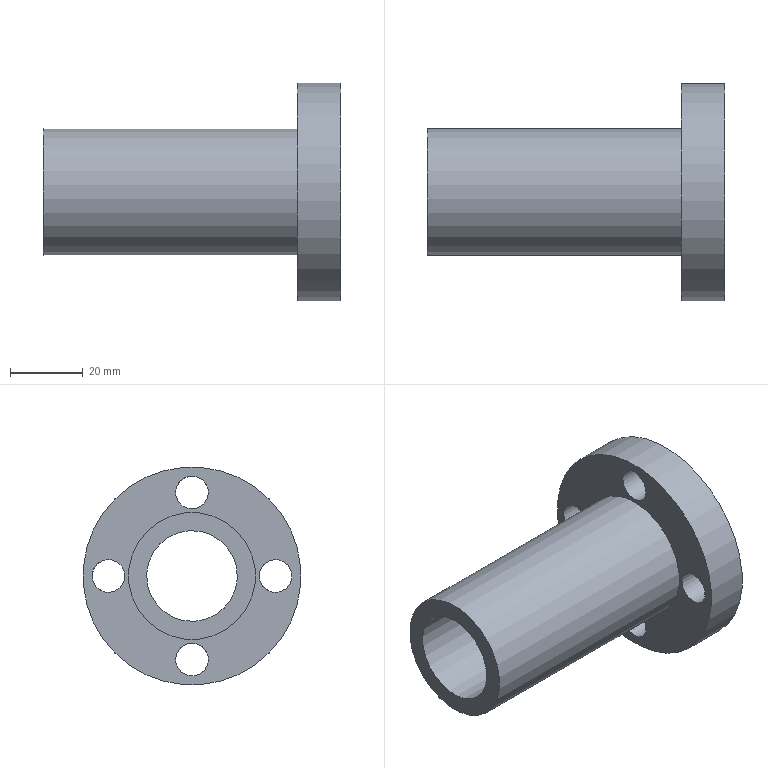Component | NX | LEADSCREW_NUT | 1 solid | 10 faces | box 82 x 60 x 60 mm | volume 57972 mm3 | cylinder 7 | plane 3 | commonest cylinder face diameters 9 x4 25 x1 60 x1 35 x1
STEP:
#1=CARTESIAN_POINT('',(0.,0.,0.));
#2=DIRECTION('',(0.,0.,1.));
#3=DIRECTION('',(1.,0.,0.));
#4=AXIS2_PLACEMENT_3D('',#1,#2,#3);
#5=CARTESIAN_POINT('',(639.189,-141.463,-1564.161));
#6=VERTEX_POINT('',#5);
#7=CARTESIAN_POINT('',(639.189,-150.302,-1573.));
#8=DIRECTION('',(-1.,0.,0.));
#9=DIRECTION('',(0.,0.7071,0.7071));
#10=AXIS2_PLACEMENT_3D('',#7,#8,#9);
#11=CIRCLE('',#10,12.5);
#12=CARTESIAN_POINT('',(639.189,-137.927,-1560.626));
#13=DIRECTION('',(1.,0.,0.));
#14=DIRECTION('',(0.,-0.7071,-0.7071));
#15=AXIS2_PLACEMENT_3D('',#12,#13,#14);
#16=PLANE('',#15);
#17=CARTESIAN_POINT('',(5.,-0.));
#18=CARTESIAN_POINT('',(5.,21.651));
#19=CARTESIAN_POINT('',(23.75,10.825));
#20=CARTESIAN_POINT('',(42.5,-0.));
#21=CARTESIAN_POINT('',(23.75,-10.825));
#22=CARTESIAN_POINT('',(5.,-21.651));
#23=CARTESIAN_POINT('',(5.,-0.));
#24=(BOUNDED_CURVE()B_SPLINE_CURVE(2,(#17,#18,#19,#20,#21,#22,#23),.UNSPECIFIED.,.T.,.F.)B_SPLINE_CURVE_WITH_KNOTS((1,2,2,2,2,1),(-2.094,0.,2.094,4.189,6.283,8.378),.UNSPECIFIED.)CURVE()GEOMETRIC_REPRESENTATION_ITEM()RATIONAL_B_SPLINE_CURVE((1.,0.5,1.,0.5,1.,0.5,1.))REPRESENTATION_ITEM(''));
#25=(GEOMETRIC_REPRESENTATION_CONTEXT(2)PARAMETRIC_REPRESENTATION_CONTEXT()REPRESENTATION_CONTEXT('',''));
#26=DEFINITIONAL_REPRESENTATION('',(#24),#25);
#27=PCURVE('',#16,#26);
#28=CARTESIAN_POINT('',(639.189,-150.302,-1573.));
#29=DIRECTION('',(-1.,0.,0.));
#30=DIRECTION('',(0.,0.7071,0.7071));
#31=AXIS2_PLACEMENT_3D('',#28,#29,#30);
#32=CYLINDRICAL_SURFACE('',#31,12.5);
#33=CARTESIAN_POINT('',(0.,0.));
#34=DIRECTION('',(1.,0.));
#35=VECTOR('',#34,1.);
#36=LINE('',#33,#35);
#37=(GEOMETRIC_REPRESENTATION_CONTEXT(2)PARAMETRIC_REPRESENTATION_CONTEXT()REPRESENTATION_CONTEXT('',''));
#38=DEFINITIONAL_REPRESENTATION('',(#36),#37);
#39=PCURVE('',#32,#38);
#40=SURFACE_CURVE('',#11,(#27,#39),.PCURVE_S1.);
#41=EDGE_CURVE('',#6,#6,#40,.T.);
#42=ORIENTED_EDGE('',*,*,#41,.F.);
#43=EDGE_LOOP('',(#42));
#44=FACE_BOUND('',#43,.T.);
#45=CARTESIAN_POINT('',(639.189,-137.927,-1560.626));
#46=VERTEX_POINT('',#45);
#47=CARTESIAN_POINT('',(639.189,-150.302,-1573.));
#48=DIRECTION('',(-1.,0.,0.));
#49=DIRECTION('',(0.,0.7071,0.7071));
#50=AXIS2_PLACEMENT_3D('',#47,#48,#49);
#51=CIRCLE('',#50,17.5);
#52=CARTESIAN_POINT('',(-0.,-0.));
#53=CARTESIAN_POINT('',(-0.,30.311));
#54=CARTESIAN_POINT('',(26.25,15.155));
#55=CARTESIAN_POINT('',(52.5,-0.));
#56=CARTESIAN_POINT('',(26.25,-15.155));
#57=CARTESIAN_POINT('',(-0.,-30.311));
#58=CARTESIAN_POINT('',(-0.,-0.));
#59=(BOUNDED_CURVE()B_SPLINE_CURVE(2,(#52,#53,#54,#55,#56,#57,#58),.UNSPECIFIED.,.T.,.F.)B_SPLINE_CURVE_WITH_KNOTS((1,2,2,2,2,1),(-2.094,0.,2.094,4.189,6.283,8.378),.UNSPECIFIED.)CURVE()GEOMETRIC_REPRESENTATION_ITEM()RATIONAL_B_SPLINE_CURVE((1.,0.5,1.,0.5,1.,0.5,1.))REPRESENTATION_ITEM(''));
#60=(GEOMETRIC_REPRESENTATION_CONTEXT(2)PARAMETRIC_REPRESENTATION_CONTEXT()REPRESENTATION_CONTEXT('',''));
#61=DEFINITIONAL_REPRESENTATION('',(#59),#60);
#62=PCURVE('',#16,#61);
#63=CARTESIAN_POINT('',(639.189,-150.302,-1573.));
#64=DIRECTION('',(-1.,0.,0.));
#65=DIRECTION('',(0.,0.7071,0.7071));
#66=AXIS2_PLACEMENT_3D('',#63,#64,#65);
#67=CYLINDRICAL_SURFACE('',#66,17.5);
#68=CARTESIAN_POINT('',(0.,0.));
#69=DIRECTION('',(1.,0.));
#70=VECTOR('',#69,1.);
#71=LINE('',#68,#70);
#72=(GEOMETRIC_REPRESENTATION_CONTEXT(2)PARAMETRIC_REPRESENTATION_CONTEXT()REPRESENTATION_CONTEXT('',''));
#73=DEFINITIONAL_REPRESENTATION('',(#71),#72);
#74=PCURVE('',#67,#73);
#75=SURFACE_CURVE('',#51,(#62,#74),.PCURVE_S1.);
#76=EDGE_CURVE('',#46,#46,#75,.T.);
#77=ORIENTED_EDGE('',*,*,#76,.T.);
#78=EDGE_LOOP('',(#77));
#79=FACE_BOUND('',#78,.T.);
#80=ADVANCED_FACE('',(#44,#79),#16,.F.);
#81=CARTESIAN_POINT('',(721.189,-141.463,-1564.161));
#82=VERTEX_POINT('',#81);
#83=CARTESIAN_POINT('',(721.189,-150.302,-1573.));
#84=DIRECTION('',(-1.,0.,0.));
#85=DIRECTION('',(0.,0.7071,0.7071));
#86=AXIS2_PLACEMENT_3D('',#83,#84,#85);
#87=CIRCLE('',#86,12.5);
#88=CARTESIAN_POINT('',(0.,-82.));
#89=DIRECTION('',(1.,0.));
#90=VECTOR('',#89,1.);
#91=LINE('',#88,#90);
#92=(GEOMETRIC_REPRESENTATION_CONTEXT(2)PARAMETRIC_REPRESENTATION_CONTEXT()REPRESENTATION_CONTEXT('',''));
#93=DEFINITIONAL_REPRESENTATION('',(#91),#92);
#94=PCURVE('',#32,#93);
#95=CARTESIAN_POINT('',(721.189,-141.463,-1564.161));
#96=DIRECTION('',(-1.,0.,0.));
#97=DIRECTION('',(0.,0.7071,0.7071));
#98=AXIS2_PLACEMENT_3D('',#95,#96,#97);
#99=PLANE('',#98);
#100=CARTESIAN_POINT('',(-12.5,-0.));
#101=DIRECTION('',(1.,0.));
#102=AXIS2_PLACEMENT_2D('',#100,#101);
#103=CIRCLE('',#102,12.5);
#104=(GEOMETRIC_REPRESENTATION_CONTEXT(2)PARAMETRIC_REPRESENTATION_CONTEXT()REPRESENTATION_CONTEXT('',''));
#105=DEFINITIONAL_REPRESENTATION('',(#103),#104);
#106=PCURVE('',#99,#105);
#107=SURFACE_CURVE('',#87,(#94,#106),.PCURVE_S1.);
#108=EDGE_CURVE('',#82,#82,#107,.T.);
#109=ORIENTED_EDGE('',*,*,#108,.T.);
#110=CARTESIAN_POINT('',(721.189,-141.463,-1564.161));
#111=CARTESIAN_POINT('',(639.189,-141.463,-1564.161));
#112=B_SPLINE_CURVE_WITH_KNOTS('',1,(#110,#111),.UNSPECIFIED.,.F.,.F.,(2,2),(-82.,0.),.PIECEWISE_BEZIER_KNOTS.);
#113=CARTESIAN_POINT('',(6.283,0.));
#114=DIRECTION('',(0.,1.));
#115=VECTOR('',#114,1.);
#116=LINE('',#113,#115);
#117=(GEOMETRIC_REPRESENTATION_CONTEXT(2)PARAMETRIC_REPRESENTATION_CONTEXT()REPRESENTATION_CONTEXT('',''));
#118=DEFINITIONAL_REPRESENTATION('',(#116),#117);
#119=PCURVE('',#32,#118);
#120=CARTESIAN_POINT('',(0.,0.));
#121=DIRECTION('',(0.,1.));
#122=VECTOR('',#121,1.);
#123=LINE('',#120,#122);
#124=(GEOMETRIC_REPRESENTATION_CONTEXT(2)PARAMETRIC_REPRESENTATION_CONTEXT()REPRESENTATION_CONTEXT('',''));
#125=DEFINITIONAL_REPRESENTATION('',(#123),#124);
#126=PCURVE('',#32,#125);
#127=SEAM_CURVE('',#112,(#119,#126),.PCURVE_S1.);
#128=EDGE_CURVE('',#82,#6,#127,.T.);
#129=ORIENTED_EDGE('',*,*,#128,.T.);
#130=ORIENTED_EDGE('',*,*,#41,.F.);
#131=ORIENTED_EDGE('',*,*,#128,.F.);
#132=EDGE_LOOP('',(#109,#129,#130,#131));
#133=FACE_BOUND('',#132,.F.);
#134=ADVANCED_FACE('',(#133),#32,.F.);
#135=CARTESIAN_POINT('',(721.189,-168.802,-1573.));
#136=VERTEX_POINT('',#135);
#137=CARTESIAN_POINT('',(721.189,-176.484,-1576.182));
#138=VERTEX_POINT('',#137);
#139=CARTESIAN_POINT('',(721.189,-173.302,-1573.));
#140=DIRECTION('',(1.,0.,0.));
#141=DIRECTION('',(0.,1.,0.));
#142=AXIS2_PLACEMENT_3D('',#139,#140,#141);
#143=CIRCLE('',#142,4.5);
#144=CARTESIAN_POINT('',(-25.581,-13.081));
#145=CARTESIAN_POINT('',(-20.07,-18.593));
#146=CARTESIAN_POINT('',(-27.599,-20.61));
#147=CARTESIAN_POINT('',(-35.127,-22.627));
#148=CARTESIAN_POINT('',(-33.11,-15.099));
#149=CARTESIAN_POINT('',(-31.093,-7.57));
#150=CARTESIAN_POINT('',(-25.581,-13.081));
#151=(BOUNDED_CURVE()B_SPLINE_CURVE(2,(#144,#145,#146,#147,#148,#149,#150),.UNSPECIFIED.,.T.,.F.)B_SPLINE_CURVE_WITH_KNOTS((1,2,2,2,2,1),(-2.094,0.,2.094,4.189,6.283,8.378),.UNSPECIFIED.)CURVE()GEOMETRIC_REPRESENTATION_ITEM()RATIONAL_B_SPLINE_CURVE((1.,0.5,1.,0.5,1.,0.5,1.))REPRESENTATION_ITEM(''));
#152=(GEOMETRIC_REPRESENTATION_CONTEXT(2)PARAMETRIC_REPRESENTATION_CONTEXT()REPRESENTATION_CONTEXT('',''));
#153=DEFINITIONAL_REPRESENTATION('',(#151),#152);
#154=PCURVE('',#99,#153);
#155=CARTESIAN_POINT('',(704.189,-173.302,-1573.));
#156=DIRECTION('',(1.,0.,0.));
#157=DIRECTION('',(0.,-0.7071,-0.7071));
#158=AXIS2_PLACEMENT_3D('',#155,#156,#157);
#159=CYLINDRICAL_SURFACE('',#158,4.5);
#160=CARTESIAN_POINT('',(2.356,17.));
#161=DIRECTION('',(1.,0.));
#162=VECTOR('',#161,1.);
#163=LINE('',#160,#162);
#164=(GEOMETRIC_REPRESENTATION_CONTEXT(2)PARAMETRIC_REPRESENTATION_CONTEXT()REPRESENTATION_CONTEXT('',''));
#165=DEFINITIONAL_REPRESENTATION('',(#163),#164);
#166=PCURVE('',#159,#165);
#167=SURFACE_CURVE('',#143,(#154,#166),.PCURVE_S1.);
#168=EDGE_CURVE('',#136,#138,#167,.T.);
#169=ORIENTED_EDGE('',*,*,#168,.F.);
#170=CARTESIAN_POINT('',(721.189,-173.302,-1573.));
#171=DIRECTION('',(1.,0.,0.));
#172=DIRECTION('',(0.,1.,0.));
#173=AXIS2_PLACEMENT_3D('',#170,#171,#172);
#174=CIRCLE('',#173,4.5);
#175=CARTESIAN_POINT('',(-25.581,-13.081));
#176=CARTESIAN_POINT('',(-20.07,-18.593));
#177=CARTESIAN_POINT('',(-27.599,-20.61));
#178=CARTESIAN_POINT('',(-35.127,-22.627));
#179=CARTESIAN_POINT('',(-33.11,-15.099));
#180=CARTESIAN_POINT('',(-31.093,-7.57));
#181=CARTESIAN_POINT('',(-25.581,-13.081));
#182=(BOUNDED_CURVE()B_SPLINE_CURVE(2,(#175,#176,#177,#178,#179,#180,#181),.UNSPECIFIED.,.T.,.F.)B_SPLINE_CURVE_WITH_KNOTS((1,2,2,2,2,1),(-2.094,0.,2.094,4.189,6.283,8.378),.UNSPECIFIED.)CURVE()GEOMETRIC_REPRESENTATION_ITEM()RATIONAL_B_SPLINE_CURVE((1.,0.5,1.,0.5,1.,0.5,1.))REPRESENTATION_ITEM(''));
#183=(GEOMETRIC_REPRESENTATION_CONTEXT(2)PARAMETRIC_REPRESENTATION_CONTEXT()REPRESENTATION_CONTEXT('',''));
#184=DEFINITIONAL_REPRESENTATION('',(#182),#183);
#185=PCURVE('',#99,#184);
#186=CARTESIAN_POINT('',(-3.927,17.));
#187=DIRECTION('',(1.,0.));
#188=VECTOR('',#187,1.);
#189=LINE('',#186,#188);
#190=(GEOMETRIC_REPRESENTATION_CONTEXT(2)PARAMETRIC_REPRESENTATION_CONTEXT()REPRESENTATION_CONTEXT('',''));
#191=DEFINITIONAL_REPRESENTATION('',(#189),#190);
#192=PCURVE('',#159,#191);
#193=SURFACE_CURVE('',#174,(#185,#192),.PCURVE_S1.);
#194=EDGE_CURVE('',#138,#136,#193,.T.);
#195=ORIENTED_EDGE('',*,*,#194,.F.);
#196=EDGE_LOOP('',(#169,#195));
#197=FACE_BOUND('',#196,.T.);
#198=CARTESIAN_POINT('',(721.189,-150.302,-1554.5));
#199=VERTEX_POINT('',#198);
#200=CARTESIAN_POINT('',(721.189,-153.484,-1553.182));
#201=VERTEX_POINT('',#200);
#202=CARTESIAN_POINT('',(721.189,-150.302,-1550.));
#203=DIRECTION('',(1.,0.,0.));
#204=DIRECTION('',(0.,0.,-1.));
#205=AXIS2_PLACEMENT_3D('',#202,#203,#204);
#206=CIRCLE('',#205,4.5);
#207=CARTESIAN_POINT('',(0.5815,-13.081));
#208=CARTESIAN_POINT('',(6.093,-7.57));
#209=CARTESIAN_POINT('',(8.11,-15.099));
#210=CARTESIAN_POINT('',(10.127,-22.627));
#211=CARTESIAN_POINT('',(2.599,-20.61));
#212=CARTESIAN_POINT('',(-4.93,-18.593));
#213=CARTESIAN_POINT('',(0.5815,-13.081));
#214=(BOUNDED_CURVE()B_SPLINE_CURVE(2,(#207,#208,#209,#210,#211,#212,#213),.UNSPECIFIED.,.T.,.F.)B_SPLINE_CURVE_WITH_KNOTS((1,2,2,2,2,1),(-2.094,0.,2.094,4.189,6.283,8.378),.UNSPECIFIED.)CURVE()GEOMETRIC_REPRESENTATION_ITEM()RATIONAL_B_SPLINE_CURVE((1.,0.5,1.,0.5,1.,0.5,1.))REPRESENTATION_ITEM(''));
#215=(GEOMETRIC_REPRESENTATION_CONTEXT(2)PARAMETRIC_REPRESENTATION_CONTEXT()REPRESENTATION_CONTEXT('',''));
#216=DEFINITIONAL_REPRESENTATION('',(#214),#215);
#217=PCURVE('',#99,#216);
#218=CARTESIAN_POINT('',(704.189,-150.302,-1550.));
#219=DIRECTION('',(1.,0.,0.));
#220=DIRECTION('',(0.,-0.7071,-0.7071));
#221=AXIS2_PLACEMENT_3D('',#218,#219,#220);
#222=CYLINDRICAL_SURFACE('',#221,4.5);
#223=CARTESIAN_POINT('',(0.7854,17.));
#224=DIRECTION('',(1.,0.));
#225=VECTOR('',#224,1.);
#226=LINE('',#223,#225);
#227=(GEOMETRIC_REPRESENTATION_CONTEXT(2)PARAMETRIC_REPRESENTATION_CONTEXT()REPRESENTATION_CONTEXT('',''));
#228=DEFINITIONAL_REPRESENTATION('',(#226),#227);
#229=PCURVE('',#222,#228);
#230=SURFACE_CURVE('',#206,(#217,#229),.PCURVE_S1.);
#231=EDGE_CURVE('',#199,#201,#230,.T.);
#232=ORIENTED_EDGE('',*,*,#231,.F.);
#233=CARTESIAN_POINT('',(721.189,-150.302,-1550.));
#234=DIRECTION('',(1.,0.,0.));
#235=DIRECTION('',(0.,0.,-1.));
#236=AXIS2_PLACEMENT_3D('',#233,#234,#235);
#237=CIRCLE('',#236,4.5);
#238=CARTESIAN_POINT('',(0.5815,-13.081));
#239=CARTESIAN_POINT('',(6.093,-7.57));
#240=CARTESIAN_POINT('',(8.11,-15.099));
#241=CARTESIAN_POINT('',(10.127,-22.627));
#242=CARTESIAN_POINT('',(2.599,-20.61));
#243=CARTESIAN_POINT('',(-4.93,-18.593));
#244=CARTESIAN_POINT('',(0.5815,-13.081));
#245=(BOUNDED_CURVE()B_SPLINE_CURVE(2,(#238,#239,#240,#241,#242,#243,#244),.UNSPECIFIED.,.T.,.F.)B_SPLINE_CURVE_WITH_KNOTS((1,2,2,2,2,1),(-2.094,0.,2.094,4.189,6.283,8.378),.UNSPECIFIED.)CURVE()GEOMETRIC_REPRESENTATION_ITEM()RATIONAL_B_SPLINE_CURVE((1.,0.5,1.,0.5,1.,0.5,1.))REPRESENTATION_ITEM(''));
#246=(GEOMETRIC_REPRESENTATION_CONTEXT(2)PARAMETRIC_REPRESENTATION_CONTEXT()REPRESENTATION_CONTEXT('',''));
#247=DEFINITIONAL_REPRESENTATION('',(#245),#246);
#248=PCURVE('',#99,#247);
#249=CARTESIAN_POINT('',(-5.498,17.));
#250=DIRECTION('',(1.,0.));
#251=VECTOR('',#250,1.);
#252=LINE('',#249,#251);
#253=(GEOMETRIC_REPRESENTATION_CONTEXT(2)PARAMETRIC_REPRESENTATION_CONTEXT()REPRESENTATION_CONTEXT('',''));
#254=DEFINITIONAL_REPRESENTATION('',(#252),#253);
#255=PCURVE('',#222,#254);
#256=SURFACE_CURVE('',#237,(#248,#255),.PCURVE_S1.);
#257=EDGE_CURVE('',#201,#199,#256,.T.);
#258=ORIENTED_EDGE('',*,*,#257,.F.);
#259=EDGE_LOOP('',(#232,#258));
#260=FACE_BOUND('',#259,.T.);
#261=CARTESIAN_POINT('',(721.189,-150.302,-1591.5));
#262=VERTEX_POINT('',#261);
#263=CARTESIAN_POINT('',(721.189,-153.484,-1599.182));
#264=VERTEX_POINT('',#263);
#265=CARTESIAN_POINT('',(721.189,-150.302,-1596.));
#266=DIRECTION('',(1.,0.,0.));
#267=DIRECTION('',(0.,-0.,1.));
#268=AXIS2_PLACEMENT_3D('',#265,#266,#267);
#269=CIRCLE('',#268,4.5);
#270=CARTESIAN_POINT('',(-25.581,13.081));
#271=CARTESIAN_POINT('',(-31.093,7.57));
#272=CARTESIAN_POINT('',(-33.11,15.099));
#273=CARTESIAN_POINT('',(-35.127,22.627));
#274=CARTESIAN_POINT('',(-27.599,20.61));
#275=CARTESIAN_POINT('',(-20.07,18.593));
#276=CARTESIAN_POINT('',(-25.581,13.081));
#277=(BOUNDED_CURVE()B_SPLINE_CURVE(2,(#270,#271,#272,#273,#274,#275,#276),.UNSPECIFIED.,.T.,.F.)B_SPLINE_CURVE_WITH_KNOTS((1,2,2,2,2,1),(-2.094,0.,2.094,4.189,6.283,8.378),.UNSPECIFIED.)CURVE()GEOMETRIC_REPRESENTATION_ITEM()RATIONAL_B_SPLINE_CURVE((1.,0.5,1.,0.5,1.,0.5,1.))REPRESENTATION_ITEM(''));
#278=(GEOMETRIC_REPRESENTATION_CONTEXT(2)PARAMETRIC_REPRESENTATION_CONTEXT()REPRESENTATION_CONTEXT('',''));
#279=DEFINITIONAL_REPRESENTATION('',(#277),#278);
#280=PCURVE('',#99,#279);
#281=CARTESIAN_POINT('',(704.189,-150.302,-1596.));
#282=DIRECTION('',(1.,0.,0.));
#283=DIRECTION('',(0.,-0.7071,-0.7071));
#284=AXIS2_PLACEMENT_3D('',#281,#282,#283);
#285=CYLINDRICAL_SURFACE('',#284,4.5);
#286=CARTESIAN_POINT('',(3.927,17.));
#287=DIRECTION('',(1.,0.));
#288=VECTOR('',#287,1.);
#289=LINE('',#286,#288);
#290=(GEOMETRIC_REPRESENTATION_CONTEXT(2)PARAMETRIC_REPRESENTATION_CONTEXT()REPRESENTATION_CONTEXT('',''));
#291=DEFINITIONAL_REPRESENTATION('',(#289),#290);
#292=PCURVE('',#285,#291);
#293=SURFACE_CURVE('',#269,(#280,#292),.PCURVE_S1.);
#294=EDGE_CURVE('',#262,#264,#293,.T.);
#295=ORIENTED_EDGE('',*,*,#294,.F.);
#296=CARTESIAN_POINT('',(721.189,-150.302,-1596.));
#297=DIRECTION('',(1.,0.,0.));
#298=DIRECTION('',(0.,-0.,1.));
#299=AXIS2_PLACEMENT_3D('',#296,#297,#298);
#300=CIRCLE('',#299,4.5);
#301=CARTESIAN_POINT('',(-25.581,13.081));
#302=CARTESIAN_POINT('',(-31.093,7.57));
#303=CARTESIAN_POINT('',(-33.11,15.099));
#304=CARTESIAN_POINT('',(-35.127,22.627));
#305=CARTESIAN_POINT('',(-27.599,20.61));
#306=CARTESIAN_POINT('',(-20.07,18.593));
#307=CARTESIAN_POINT('',(-25.581,13.081));
#308=(BOUNDED_CURVE()B_SPLINE_CURVE(2,(#301,#302,#303,#304,#305,#306,#307),.UNSPECIFIED.,.T.,.F.)B_SPLINE_CURVE_WITH_KNOTS((1,2,2,2,2,1),(-2.094,0.,2.094,4.189,6.283,8.378),.UNSPECIFIED.)CURVE()GEOMETRIC_REPRESENTATION_ITEM()RATIONAL_B_SPLINE_CURVE((1.,0.5,1.,0.5,1.,0.5,1.))REPRESENTATION_ITEM(''));
#309=(GEOMETRIC_REPRESENTATION_CONTEXT(2)PARAMETRIC_REPRESENTATION_CONTEXT()REPRESENTATION_CONTEXT('',''));
#310=DEFINITIONAL_REPRESENTATION('',(#308),#309);
#311=PCURVE('',#99,#310);
#312=CARTESIAN_POINT('',(-2.356,17.));
#313=DIRECTION('',(1.,0.));
#314=VECTOR('',#313,1.);
#315=LINE('',#312,#314);
#316=(GEOMETRIC_REPRESENTATION_CONTEXT(2)PARAMETRIC_REPRESENTATION_CONTEXT()REPRESENTATION_CONTEXT('',''));
#317=DEFINITIONAL_REPRESENTATION('',(#315),#316);
#318=PCURVE('',#285,#317);
#319=SURFACE_CURVE('',#300,(#311,#318),.PCURVE_S1.);
#320=EDGE_CURVE('',#264,#262,#319,.T.);
#321=ORIENTED_EDGE('',*,*,#320,.F.);
#322=EDGE_LOOP('',(#295,#321));
#323=FACE_BOUND('',#322,.T.);
#324=CARTESIAN_POINT('',(721.189,-131.802,-1573.));
#325=VERTEX_POINT('',#324);
#326=CARTESIAN_POINT('',(721.189,-130.484,-1576.182));
#327=VERTEX_POINT('',#326);
#328=CARTESIAN_POINT('',(721.189,-127.302,-1573.));
#329=DIRECTION('',(1.,0.,0.));
#330=DIRECTION('',(0.,-1.,0.));
#331=AXIS2_PLACEMENT_3D('',#328,#329,#330);
#332=CIRCLE('',#331,4.5);
#333=CARTESIAN_POINT('',(0.5815,13.081));
#334=CARTESIAN_POINT('',(-4.93,18.593));
#335=CARTESIAN_POINT('',(2.599,20.61));
#336=CARTESIAN_POINT('',(10.127,22.627));
#337=CARTESIAN_POINT('',(8.11,15.099));
#338=CARTESIAN_POINT('',(6.093,7.57));
#339=CARTESIAN_POINT('',(0.5815,13.081));
#340=(BOUNDED_CURVE()B_SPLINE_CURVE(2,(#333,#334,#335,#336,#337,#338,#339),.UNSPECIFIED.,.T.,.F.)B_SPLINE_CURVE_WITH_KNOTS((1,2,2,2,2,1),(-2.094,0.,2.094,4.189,6.283,8.378),.UNSPECIFIED.)CURVE()GEOMETRIC_REPRESENTATION_ITEM()RATIONAL_B_SPLINE_CURVE((1.,0.5,1.,0.5,1.,0.5,1.))REPRESENTATION_ITEM(''));
#341=(GEOMETRIC_REPRESENTATION_CONTEXT(2)PARAMETRIC_REPRESENTATION_CONTEXT()REPRESENTATION_CONTEXT('',''));
#342=DEFINITIONAL_REPRESENTATION('',(#340),#341);
#343=PCURVE('',#99,#342);
#344=CARTESIAN_POINT('',(704.189,-127.302,-1573.));
#345=DIRECTION('',(1.,0.,0.));
#346=DIRECTION('',(0.,-0.7071,-0.7071));
#347=AXIS2_PLACEMENT_3D('',#344,#345,#346);
#348=CYLINDRICAL_SURFACE('',#347,4.5);
#349=CARTESIAN_POINT('',(5.498,17.));
#350=DIRECTION('',(1.,0.));
#351=VECTOR('',#350,1.);
#352=LINE('',#349,#351);
#353=(GEOMETRIC_REPRESENTATION_CONTEXT(2)PARAMETRIC_REPRESENTATION_CONTEXT()REPRESENTATION_CONTEXT('',''));
#354=DEFINITIONAL_REPRESENTATION('',(#352),#353);
#355=PCURVE('',#348,#354);
#356=SURFACE_CURVE('',#332,(#343,#355),.PCURVE_S1.);
#357=EDGE_CURVE('',#325,#327,#356,.T.);
#358=ORIENTED_EDGE('',*,*,#357,.F.);
#359=CARTESIAN_POINT('',(721.189,-127.302,-1573.));
#360=DIRECTION('',(1.,0.,0.));
#361=DIRECTION('',(0.,-1.,0.));
#362=AXIS2_PLACEMENT_3D('',#359,#360,#361);
#363=CIRCLE('',#362,4.5);
#364=CARTESIAN_POINT('',(0.5815,13.081));
#365=CARTESIAN_POINT('',(-4.93,18.593));
#366=CARTESIAN_POINT('',(2.599,20.61));
#367=CARTESIAN_POINT('',(10.127,22.627));
#368=CARTESIAN_POINT('',(8.11,15.099));
#369=CARTESIAN_POINT('',(6.093,7.57));
#370=CARTESIAN_POINT('',(0.5815,13.081));
#371=(BOUNDED_CURVE()B_SPLINE_CURVE(2,(#364,#365,#366,#367,#368,#369,#370),.UNSPECIFIED.,.T.,.F.)B_SPLINE_CURVE_WITH_KNOTS((1,2,2,2,2,1),(-2.094,0.,2.094,4.189,6.283,8.378),.UNSPECIFIED.)CURVE()GEOMETRIC_REPRESENTATION_ITEM()RATIONAL_B_SPLINE_CURVE((1.,0.5,1.,0.5,1.,0.5,1.))REPRESENTATION_ITEM(''));
#372=(GEOMETRIC_REPRESENTATION_CONTEXT(2)PARAMETRIC_REPRESENTATION_CONTEXT()REPRESENTATION_CONTEXT('',''));
#373=DEFINITIONAL_REPRESENTATION('',(#371),#372);
#374=PCURVE('',#99,#373);
#375=CARTESIAN_POINT('',(-0.7854,17.));
#376=DIRECTION('',(1.,0.));
#377=VECTOR('',#376,1.);
#378=LINE('',#375,#377);
#379=(GEOMETRIC_REPRESENTATION_CONTEXT(2)PARAMETRIC_REPRESENTATION_CONTEXT()REPRESENTATION_CONTEXT('',''));
#380=DEFINITIONAL_REPRESENTATION('',(#378),#379);
#381=PCURVE('',#348,#380);
#382=SURFACE_CURVE('',#363,(#374,#381),.PCURVE_S1.);
#383=EDGE_CURVE('',#327,#325,#382,.T.);
#384=ORIENTED_EDGE('',*,*,#383,.F.);
#385=EDGE_LOOP('',(#358,#384));
#386=FACE_BOUND('',#385,.T.);
#387=CARTESIAN_POINT('',(721.189,-129.088,-1551.787));
#388=VERTEX_POINT('',#387);
#389=CARTESIAN_POINT('',(721.189,-150.302,-1573.));
#390=DIRECTION('',(-1.,0.,0.));
#391=DIRECTION('',(0.,0.7071,0.7071));
#392=AXIS2_PLACEMENT_3D('',#389,#390,#391);
#393=CIRCLE('',#392,30.);
#394=CARTESIAN_POINT('',(-12.5,-0.));
#395=DIRECTION('',(1.,0.));
#396=AXIS2_PLACEMENT_2D('',#394,#395);
#397=CIRCLE('',#396,30.);
#398=(GEOMETRIC_REPRESENTATION_CONTEXT(2)PARAMETRIC_REPRESENTATION_CONTEXT()REPRESENTATION_CONTEXT('',''));
#399=DEFINITIONAL_REPRESENTATION('',(#397),#398);
#400=PCURVE('',#99,#399);
#401=CARTESIAN_POINT('',(639.189,-150.302,-1573.));
#402=DIRECTION('',(-1.,0.,0.));
#403=DIRECTION('',(0.,0.7071,0.7071));
#404=AXIS2_PLACEMENT_3D('',#401,#402,#403);
#405=CYLINDRICAL_SURFACE('',#404,30.);
#406=CARTESIAN_POINT('',(0.,-82.));
#407=DIRECTION('',(1.,0.));
#408=VECTOR('',#407,1.);
#409=LINE('',#406,#408);
#410=(GEOMETRIC_REPRESENTATION_CONTEXT(2)PARAMETRIC_REPRESENTATION_CONTEXT()REPRESENTATION_CONTEXT('',''));
#411=DEFINITIONAL_REPRESENTATION('',(#409),#410);
#412=PCURVE('',#405,#411);
#413=SURFACE_CURVE('',#393,(#400,#412),.PCURVE_S1.);
#414=EDGE_CURVE('',#388,#388,#413,.T.);
#415=ORIENTED_EDGE('',*,*,#414,.F.);
#416=EDGE_LOOP('',(#415));
#417=FACE_BOUND('',#416,.T.);
#418=ORIENTED_EDGE('',*,*,#108,.T.);
#419=EDGE_LOOP('',(#418));
#420=FACE_BOUND('',#419,.T.);
#421=ADVANCED_FACE('',(#197,#260,#323,#386,#417,#420),#99,.F.);
#422=CARTESIAN_POINT('',(709.189,-129.088,-1551.787));
#423=VERTEX_POINT('',#422);
#424=CARTESIAN_POINT('',(709.189,-150.302,-1573.));
#425=DIRECTION('',(-1.,0.,0.));
#426=DIRECTION('',(0.,0.7071,0.7071));
#427=AXIS2_PLACEMENT_3D('',#424,#425,#426);
#428=CIRCLE('',#427,30.);
#429=CARTESIAN_POINT('',(0.,-70.));
#430=DIRECTION('',(1.,0.));
#431=VECTOR('',#430,1.);
#432=LINE('',#429,#431);
#433=(GEOMETRIC_REPRESENTATION_CONTEXT(2)PARAMETRIC_REPRESENTATION_CONTEXT()REPRESENTATION_CONTEXT('',''));
#434=DEFINITIONAL_REPRESENTATION('',(#432),#433);
#435=PCURVE('',#405,#434);
#436=CARTESIAN_POINT('',(709.189,-129.088,-1551.787));
#437=DIRECTION('',(1.,0.,0.));
#438=DIRECTION('',(0.,-0.7071,-0.7071));
#439=AXIS2_PLACEMENT_3D('',#436,#437,#438);
#440=PLANE('',#439);
#441=CARTESIAN_POINT('',(0.,0.));
#442=CARTESIAN_POINT('',(0.,51.962));
#443=CARTESIAN_POINT('',(45.,25.981));
#444=CARTESIAN_POINT('',(90.,0.));
#445=CARTESIAN_POINT('',(45.,-25.981));
#446=CARTESIAN_POINT('',(0.,-51.962));
#447=CARTESIAN_POINT('',(0.,0.));
#448=(BOUNDED_CURVE()B_SPLINE_CURVE(2,(#441,#442,#443,#444,#445,#446,#447),.UNSPECIFIED.,.T.,.F.)B_SPLINE_CURVE_WITH_KNOTS((1,2,2,2,2,1),(-2.094,0.,2.094,4.189,6.283,8.378),.UNSPECIFIED.)CURVE()GEOMETRIC_REPRESENTATION_ITEM()RATIONAL_B_SPLINE_CURVE((1.,0.5,1.,0.5,1.,0.5,1.))REPRESENTATION_ITEM(''));
#449=(GEOMETRIC_REPRESENTATION_CONTEXT(2)PARAMETRIC_REPRESENTATION_CONTEXT()REPRESENTATION_CONTEXT('',''));
#450=DEFINITIONAL_REPRESENTATION('',(#448),#449);
#451=PCURVE('',#440,#450);
#452=SURFACE_CURVE('',#428,(#435,#451),.PCURVE_S1.);
#453=EDGE_CURVE('',#423,#423,#452,.T.);
#454=ORIENTED_EDGE('',*,*,#453,.F.);
#455=CARTESIAN_POINT('',(721.189,-129.088,-1551.787));
#456=CARTESIAN_POINT('',(709.189,-129.088,-1551.787));
#457=B_SPLINE_CURVE_WITH_KNOTS('',1,(#455,#456),.UNSPECIFIED.,.F.,.F.,(2,2),(-82.,-70.),.PIECEWISE_BEZIER_KNOTS.);
#458=CARTESIAN_POINT('',(0.,0.));
#459=DIRECTION('',(0.,1.));
#460=VECTOR('',#459,1.);
#461=LINE('',#458,#460);
#462=(GEOMETRIC_REPRESENTATION_CONTEXT(2)PARAMETRIC_REPRESENTATION_CONTEXT()REPRESENTATION_CONTEXT('',''));
#463=DEFINITIONAL_REPRESENTATION('',(#461),#462);
#464=PCURVE('',#405,#463);
#465=CARTESIAN_POINT('',(6.283,0.));
#466=DIRECTION('',(0.,1.));
#467=VECTOR('',#466,1.);
#468=LINE('',#465,#467);
#469=(GEOMETRIC_REPRESENTATION_CONTEXT(2)PARAMETRIC_REPRESENTATION_CONTEXT()REPRESENTATION_CONTEXT('',''));
#470=DEFINITIONAL_REPRESENTATION('',(#468),#469);
#471=PCURVE('',#405,#470);
#472=SEAM_CURVE('',#457,(#464,#471),.PCURVE_S1.);
#473=EDGE_CURVE('',#388,#423,#472,.T.);
#474=ORIENTED_EDGE('',*,*,#473,.F.);
#475=ORIENTED_EDGE('',*,*,#414,.T.);
#476=ORIENTED_EDGE('',*,*,#473,.T.);
#477=EDGE_LOOP('',(#454,#474,#475,#476));
#478=FACE_BOUND('',#477,.T.);
#479=ADVANCED_FACE('',(#478),#405,.T.);
#480=CARTESIAN_POINT('',(709.189,-176.484,-1576.182));
#481=VERTEX_POINT('',#480);
#482=CARTESIAN_POINT('',(709.189,-173.302,-1573.));
#483=DIRECTION('',(1.,0.,0.));
#484=DIRECTION('',(0.,-0.7071,-0.7071));
#485=AXIS2_PLACEMENT_3D('',#482,#483,#484);
#486=CIRCLE('',#485,4.5);
#487=CARTESIAN_POINT('',(46.263,-16.263));
#488=DIRECTION('',(1.,-0.));
#489=AXIS2_PLACEMENT_2D('',#487,#488);
#490=CIRCLE('',#489,4.5);
#491=(GEOMETRIC_REPRESENTATION_CONTEXT(2)PARAMETRIC_REPRESENTATION_CONTEXT()REPRESENTATION_CONTEXT('',''));
#492=DEFINITIONAL_REPRESENTATION('',(#490),#491);
#493=PCURVE('',#440,#492);
#494=CARTESIAN_POINT('',(0.,5.));
#495=DIRECTION('',(1.,0.));
#496=VECTOR('',#495,1.);
#497=LINE('',#494,#496);
#498=(GEOMETRIC_REPRESENTATION_CONTEXT(2)PARAMETRIC_REPRESENTATION_CONTEXT()REPRESENTATION_CONTEXT('',''));
#499=DEFINITIONAL_REPRESENTATION('',(#497),#498);
#500=PCURVE('',#159,#499);
#501=SURFACE_CURVE('',#486,(#493,#500),.PCURVE_S1.);
#502=EDGE_CURVE('',#481,#481,#501,.T.);
#503=ORIENTED_EDGE('',*,*,#502,.T.);
#504=EDGE_LOOP('',(#503));
#505=FACE_BOUND('',#504,.T.);
#506=CARTESIAN_POINT('',(709.189,-153.484,-1553.182));
#507=VERTEX_POINT('',#506);
#508=CARTESIAN_POINT('',(709.189,-150.302,-1550.));
#509=DIRECTION('',(1.,0.,0.));
#510=DIRECTION('',(0.,-0.7071,-0.7071));
#511=AXIS2_PLACEMENT_3D('',#508,#509,#510);
#512=CIRCLE('',#511,4.5);
#513=CARTESIAN_POINT('',(13.737,-16.263));
#514=DIRECTION('',(1.,-0.));
#515=AXIS2_PLACEMENT_2D('',#513,#514);
#516=CIRCLE('',#515,4.5);
#517=(GEOMETRIC_REPRESENTATION_CONTEXT(2)PARAMETRIC_REPRESENTATION_CONTEXT()REPRESENTATION_CONTEXT('',''));
#518=DEFINITIONAL_REPRESENTATION('',(#516),#517);
#519=PCURVE('',#440,#518);
#520=CARTESIAN_POINT('',(0.,5.));
#521=DIRECTION('',(1.,0.));
#522=VECTOR('',#521,1.);
#523=LINE('',#520,#522);
#524=(GEOMETRIC_REPRESENTATION_CONTEXT(2)PARAMETRIC_REPRESENTATION_CONTEXT()REPRESENTATION_CONTEXT('',''));
#525=DEFINITIONAL_REPRESENTATION('',(#523),#524);
#526=PCURVE('',#222,#525);
#527=SURFACE_CURVE('',#512,(#519,#526),.PCURVE_S1.);
#528=EDGE_CURVE('',#507,#507,#527,.T.);
#529=ORIENTED_EDGE('',*,*,#528,.T.);
#530=EDGE_LOOP('',(#529));
#531=FACE_BOUND('',#530,.T.);
#532=CARTESIAN_POINT('',(709.189,-153.484,-1599.182));
#533=VERTEX_POINT('',#532);
#534=CARTESIAN_POINT('',(709.189,-150.302,-1596.));
#535=DIRECTION('',(1.,0.,0.));
#536=DIRECTION('',(0.,-0.7071,-0.7071));
#537=AXIS2_PLACEMENT_3D('',#534,#535,#536);
#538=CIRCLE('',#537,4.5);
#539=CARTESIAN_POINT('',(46.263,16.263));
#540=DIRECTION('',(1.,-0.));
#541=AXIS2_PLACEMENT_2D('',#539,#540);
#542=CIRCLE('',#541,4.5);
#543=(GEOMETRIC_REPRESENTATION_CONTEXT(2)PARAMETRIC_REPRESENTATION_CONTEXT()REPRESENTATION_CONTEXT('',''));
#544=DEFINITIONAL_REPRESENTATION('',(#542),#543);
#545=PCURVE('',#440,#544);
#546=CARTESIAN_POINT('',(0.,5.));
#547=DIRECTION('',(1.,0.));
#548=VECTOR('',#547,1.);
#549=LINE('',#546,#548);
#550=(GEOMETRIC_REPRESENTATION_CONTEXT(2)PARAMETRIC_REPRESENTATION_CONTEXT()REPRESENTATION_CONTEXT('',''));
#551=DEFINITIONAL_REPRESENTATION('',(#549),#550);
#552=PCURVE('',#285,#551);
#553=SURFACE_CURVE('',#538,(#545,#552),.PCURVE_S1.);
#554=EDGE_CURVE('',#533,#533,#553,.T.);
#555=ORIENTED_EDGE('',*,*,#554,.T.);
#556=EDGE_LOOP('',(#555));
#557=FACE_BOUND('',#556,.T.);
#558=CARTESIAN_POINT('',(709.189,-130.484,-1576.182));
#559=VERTEX_POINT('',#558);
#560=CARTESIAN_POINT('',(709.189,-127.302,-1573.));
#561=DIRECTION('',(1.,0.,0.));
#562=DIRECTION('',(0.,-0.7071,-0.7071));
#563=AXIS2_PLACEMENT_3D('',#560,#561,#562);
#564=CIRCLE('',#563,4.5);
#565=CARTESIAN_POINT('',(13.737,16.263));
#566=DIRECTION('',(1.,-0.));
#567=AXIS2_PLACEMENT_2D('',#565,#566);
#568=CIRCLE('',#567,4.5);
#569=(GEOMETRIC_REPRESENTATION_CONTEXT(2)PARAMETRIC_REPRESENTATION_CONTEXT()REPRESENTATION_CONTEXT('',''));
#570=DEFINITIONAL_REPRESENTATION('',(#568),#569);
#571=PCURVE('',#440,#570);
#572=CARTESIAN_POINT('',(0.,5.));
#573=DIRECTION('',(1.,0.));
#574=VECTOR('',#573,1.);
#575=LINE('',#572,#574);
#576=(GEOMETRIC_REPRESENTATION_CONTEXT(2)PARAMETRIC_REPRESENTATION_CONTEXT()REPRESENTATION_CONTEXT('',''));
#577=DEFINITIONAL_REPRESENTATION('',(#575),#576);
#578=PCURVE('',#348,#577);
#579=SURFACE_CURVE('',#564,(#571,#578),.PCURVE_S1.);
#580=EDGE_CURVE('',#559,#559,#579,.T.);
#581=ORIENTED_EDGE('',*,*,#580,.T.);
#582=EDGE_LOOP('',(#581));
#583=FACE_BOUND('',#582,.T.);
#584=CARTESIAN_POINT('',(709.189,-137.927,-1560.626));
#585=VERTEX_POINT('',#584);
#586=CARTESIAN_POINT('',(709.189,-150.302,-1573.));
#587=DIRECTION('',(-1.,0.,0.));
#588=DIRECTION('',(0.,0.7071,0.7071));
#589=AXIS2_PLACEMENT_3D('',#586,#587,#588);
#590=CIRCLE('',#589,17.5);
#591=CARTESIAN_POINT('',(12.5,0.));
#592=CARTESIAN_POINT('',(12.5,30.311));
#593=CARTESIAN_POINT('',(38.75,15.155));
#594=CARTESIAN_POINT('',(65.,0.));
#595=CARTESIAN_POINT('',(38.75,-15.155));
#596=CARTESIAN_POINT('',(12.5,-30.311));
#597=CARTESIAN_POINT('',(12.5,0.));
#598=(BOUNDED_CURVE()B_SPLINE_CURVE(2,(#591,#592,#593,#594,#595,#596,#597),.UNSPECIFIED.,.T.,.F.)B_SPLINE_CURVE_WITH_KNOTS((1,2,2,2,2,1),(-2.094,0.,2.094,4.189,6.283,8.378),.UNSPECIFIED.)CURVE()GEOMETRIC_REPRESENTATION_ITEM()RATIONAL_B_SPLINE_CURVE((1.,0.5,1.,0.5,1.,0.5,1.))REPRESENTATION_ITEM(''));
#599=(GEOMETRIC_REPRESENTATION_CONTEXT(2)PARAMETRIC_REPRESENTATION_CONTEXT()REPRESENTATION_CONTEXT('',''));
#600=DEFINITIONAL_REPRESENTATION('',(#598),#599);
#601=PCURVE('',#440,#600);
#602=CARTESIAN_POINT('',(0.,-70.));
#603=DIRECTION('',(1.,0.));
#604=VECTOR('',#603,1.);
#605=LINE('',#602,#604);
#606=(GEOMETRIC_REPRESENTATION_CONTEXT(2)PARAMETRIC_REPRESENTATION_CONTEXT()REPRESENTATION_CONTEXT('',''));
#607=DEFINITIONAL_REPRESENTATION('',(#605),#606);
#608=PCURVE('',#67,#607);
#609=SURFACE_CURVE('',#590,(#601,#608),.PCURVE_S1.);
#610=EDGE_CURVE('',#585,#585,#609,.T.);
#611=ORIENTED_EDGE('',*,*,#610,.F.);
#612=EDGE_LOOP('',(#611));
#613=FACE_BOUND('',#612,.T.);
#614=ORIENTED_EDGE('',*,*,#453,.T.);
#615=EDGE_LOOP('',(#614));
#616=FACE_BOUND('',#615,.T.);
#617=ADVANCED_FACE('',(#505,#531,#557,#583,#613,#616),#440,.F.);
#618=ORIENTED_EDGE('',*,*,#76,.F.);
#619=CARTESIAN_POINT('',(709.189,-137.927,-1560.626));
#620=CARTESIAN_POINT('',(639.189,-137.927,-1560.626));
#621=B_SPLINE_CURVE_WITH_KNOTS('',1,(#619,#620),.UNSPECIFIED.,.F.,.F.,(2,2),(-70.,0.),.PIECEWISE_BEZIER_KNOTS.);
#622=CARTESIAN_POINT('',(0.,0.));
#623=DIRECTION('',(0.,1.));
#624=VECTOR('',#623,1.);
#625=LINE('',#622,#624);
#626=(GEOMETRIC_REPRESENTATION_CONTEXT(2)PARAMETRIC_REPRESENTATION_CONTEXT()REPRESENTATION_CONTEXT('',''));
#627=DEFINITIONAL_REPRESENTATION('',(#625),#626);
#628=PCURVE('',#67,#627);
#629=CARTESIAN_POINT('',(6.283,0.));
#630=DIRECTION('',(0.,1.));
#631=VECTOR('',#630,1.);
#632=LINE('',#629,#631);
#633=(GEOMETRIC_REPRESENTATION_CONTEXT(2)PARAMETRIC_REPRESENTATION_CONTEXT()REPRESENTATION_CONTEXT('',''));
#634=DEFINITIONAL_REPRESENTATION('',(#632),#633);
#635=PCURVE('',#67,#634);
#636=SEAM_CURVE('',#621,(#628,#635),.PCURVE_S1.);
#637=EDGE_CURVE('',#585,#46,#636,.T.);
#638=ORIENTED_EDGE('',*,*,#637,.F.);
#639=ORIENTED_EDGE('',*,*,#610,.T.);
#640=ORIENTED_EDGE('',*,*,#637,.T.);
#641=EDGE_LOOP('',(#618,#638,#639,#640));
#642=FACE_BOUND('',#641,.T.);
#643=ADVANCED_FACE('',(#642),#67,.T.);
#644=ORIENTED_EDGE('',*,*,#383,.F.);
#645=CARTESIAN_POINT('',(709.189,-130.484,-1576.182));
#646=CARTESIAN_POINT('',(721.189,-130.484,-1576.182));
#647=B_SPLINE_CURVE_WITH_KNOTS('',1,(#645,#646),.UNSPECIFIED.,.F.,.F.,(2,2),(5.,17.),.PIECEWISE_BEZIER_KNOTS.);
#648=CARTESIAN_POINT('',(0.,0.));
#649=DIRECTION('',(0.,1.));
#650=VECTOR('',#649,1.);
#651=LINE('',#648,#650);
#652=(GEOMETRIC_REPRESENTATION_CONTEXT(2)PARAMETRIC_REPRESENTATION_CONTEXT()REPRESENTATION_CONTEXT('',''));
#653=DEFINITIONAL_REPRESENTATION('',(#651),#652);
#654=PCURVE('',#348,#653);
#655=CARTESIAN_POINT('',(6.283,0.));
#656=DIRECTION('',(0.,1.));
#657=VECTOR('',#656,1.);
#658=LINE('',#655,#657);
#659=(GEOMETRIC_REPRESENTATION_CONTEXT(2)PARAMETRIC_REPRESENTATION_CONTEXT()REPRESENTATION_CONTEXT('',''));
#660=DEFINITIONAL_REPRESENTATION('',(#658),#659);
#661=PCURVE('',#348,#660);
#662=SEAM_CURVE('',#647,(#654,#661),.PCURVE_S1.);
#663=EDGE_CURVE('',#559,#327,#662,.T.);
#664=ORIENTED_EDGE('',*,*,#663,.F.);
#665=ORIENTED_EDGE('',*,*,#580,.T.);
#666=ORIENTED_EDGE('',*,*,#663,.T.);
#667=ORIENTED_EDGE('',*,*,#357,.F.);
#668=EDGE_LOOP('',(#644,#664,#665,#666,#667));
#669=FACE_BOUND('',#668,.F.);
#670=ADVANCED_FACE('',(#669),#348,.F.);
#671=ORIENTED_EDGE('',*,*,#320,.F.);
#672=CARTESIAN_POINT('',(709.189,-153.484,-1599.182));
#673=CARTESIAN_POINT('',(721.189,-153.484,-1599.182));
#674=B_SPLINE_CURVE_WITH_KNOTS('',1,(#672,#673),.UNSPECIFIED.,.F.,.F.,(2,2),(5.,17.),.PIECEWISE_BEZIER_KNOTS.);
#675=CARTESIAN_POINT('',(0.,0.));
#676=DIRECTION('',(0.,1.));
#677=VECTOR('',#676,1.);
#678=LINE('',#675,#677);
#679=(GEOMETRIC_REPRESENTATION_CONTEXT(2)PARAMETRIC_REPRESENTATION_CONTEXT()REPRESENTATION_CONTEXT('',''));
#680=DEFINITIONAL_REPRESENTATION('',(#678),#679);
#681=PCURVE('',#285,#680);
#682=CARTESIAN_POINT('',(6.283,0.));
#683=DIRECTION('',(0.,1.));
#684=VECTOR('',#683,1.);
#685=LINE('',#682,#684);
#686=(GEOMETRIC_REPRESENTATION_CONTEXT(2)PARAMETRIC_REPRESENTATION_CONTEXT()REPRESENTATION_CONTEXT('',''));
#687=DEFINITIONAL_REPRESENTATION('',(#685),#686);
#688=PCURVE('',#285,#687);
#689=SEAM_CURVE('',#674,(#681,#688),.PCURVE_S1.);
#690=EDGE_CURVE('',#533,#264,#689,.T.);
#691=ORIENTED_EDGE('',*,*,#690,.F.);
#692=ORIENTED_EDGE('',*,*,#554,.T.);
#693=ORIENTED_EDGE('',*,*,#690,.T.);
#694=ORIENTED_EDGE('',*,*,#294,.F.);
#695=EDGE_LOOP('',(#671,#691,#692,#693,#694));
#696=FACE_BOUND('',#695,.F.);
#697=ADVANCED_FACE('',(#696),#285,.F.);
#698=ORIENTED_EDGE('',*,*,#257,.F.);
#699=CARTESIAN_POINT('',(709.189,-153.484,-1553.182));
#700=CARTESIAN_POINT('',(721.189,-153.484,-1553.182));
#701=B_SPLINE_CURVE_WITH_KNOTS('',1,(#699,#700),.UNSPECIFIED.,.F.,.F.,(2,2),(5.,17.),.PIECEWISE_BEZIER_KNOTS.);
#702=CARTESIAN_POINT('',(0.,0.));
#703=DIRECTION('',(0.,1.));
#704=VECTOR('',#703,1.);
#705=LINE('',#702,#704);
#706=(GEOMETRIC_REPRESENTATION_CONTEXT(2)PARAMETRIC_REPRESENTATION_CONTEXT()REPRESENTATION_CONTEXT('',''));
#707=DEFINITIONAL_REPRESENTATION('',(#705),#706);
#708=PCURVE('',#222,#707);
#709=CARTESIAN_POINT('',(6.283,0.));
#710=DIRECTION('',(0.,1.));
#711=VECTOR('',#710,1.);
#712=LINE('',#709,#711);
#713=(GEOMETRIC_REPRESENTATION_CONTEXT(2)PARAMETRIC_REPRESENTATION_CONTEXT()REPRESENTATION_CONTEXT('',''));
#714=DEFINITIONAL_REPRESENTATION('',(#712),#713);
#715=PCURVE('',#222,#714);
#716=SEAM_CURVE('',#701,(#708,#715),.PCURVE_S1.);
#717=EDGE_CURVE('',#507,#201,#716,.T.);
#718=ORIENTED_EDGE('',*,*,#717,.F.);
#719=ORIENTED_EDGE('',*,*,#528,.T.);
#720=ORIENTED_EDGE('',*,*,#717,.T.);
#721=ORIENTED_EDGE('',*,*,#231,.F.);
#722=EDGE_LOOP('',(#698,#718,#719,#720,#721));
#723=FACE_BOUND('',#722,.F.);
#724=ADVANCED_FACE('',(#723),#222,.F.);
#725=ORIENTED_EDGE('',*,*,#194,.F.);
#726=CARTESIAN_POINT('',(709.189,-176.484,-1576.182));
#727=CARTESIAN_POINT('',(721.189,-176.484,-1576.182));
#728=B_SPLINE_CURVE_WITH_KNOTS('',1,(#726,#727),.UNSPECIFIED.,.F.,.F.,(2,2),(5.,17.),.PIECEWISE_BEZIER_KNOTS.);
#729=CARTESIAN_POINT('',(0.,0.));
#730=DIRECTION('',(0.,1.));
#731=VECTOR('',#730,1.);
#732=LINE('',#729,#731);
#733=(GEOMETRIC_REPRESENTATION_CONTEXT(2)PARAMETRIC_REPRESENTATION_CONTEXT()REPRESENTATION_CONTEXT('',''));
#734=DEFINITIONAL_REPRESENTATION('',(#732),#733);
#735=PCURVE('',#159,#734);
#736=CARTESIAN_POINT('',(6.283,0.));
#737=DIRECTION('',(0.,1.));
#738=VECTOR('',#737,1.);
#739=LINE('',#736,#738);
#740=(GEOMETRIC_REPRESENTATION_CONTEXT(2)PARAMETRIC_REPRESENTATION_CONTEXT()REPRESENTATION_CONTEXT('',''));
#741=DEFINITIONAL_REPRESENTATION('',(#739),#740);
#742=PCURVE('',#159,#741);
#743=SEAM_CURVE('',#728,(#735,#742),.PCURVE_S1.);
#744=EDGE_CURVE('',#481,#138,#743,.T.);
#745=ORIENTED_EDGE('',*,*,#744,.F.);
#746=ORIENTED_EDGE('',*,*,#502,.T.);
#747=ORIENTED_EDGE('',*,*,#744,.T.);
#748=ORIENTED_EDGE('',*,*,#168,.F.);
#749=EDGE_LOOP('',(#725,#745,#746,#747,#748));
#750=FACE_BOUND('',#749,.F.);
#751=ADVANCED_FACE('',(#750),#159,.F.);
#752=CLOSED_SHELL('',(#80,#134,#421,#479,#617,#643,#670,#697,#724,#751));
#753=MANIFOLD_SOLID_BREP('',#752);
#754=(LENGTH_UNIT()NAMED_UNIT(*)SI_UNIT(.MILLI.,.METRE.));
#755=UNCERTAINTY_MEASURE_WITH_UNIT(LENGTH_MEASURE(0.000005),#754,'','');
#756=(NAMED_UNIT(*)PLANE_ANGLE_UNIT()SI_UNIT($,.RADIAN.));
#757=(NAMED_UNIT(*)SI_UNIT($,.STERADIAN.)SOLID_ANGLE_UNIT());
#758=(GEOMETRIC_REPRESENTATION_CONTEXT(3)GLOBAL_UNCERTAINTY_ASSIGNED_CONTEXT((#755))GLOBAL_UNIT_ASSIGNED_CONTEXT((#754,#756,#757))REPRESENTATION_CONTEXT('',''));
#759=ADVANCED_BREP_SHAPE_REPRESENTATION('',(#4,#753),#758);